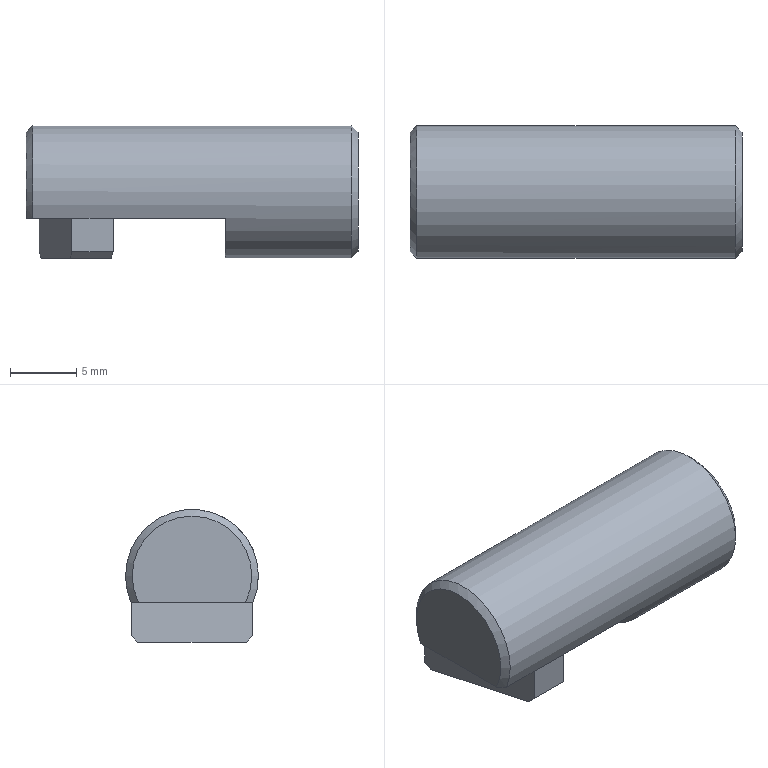Component | NX | GUIDE_PILLAR_B | 1 solid | 15 faces | box 25 x 10 x 10 mm | volume 1745 mm3 | plane 12 | cone 2 | cylinder 1 | commonest cylinder face diameters 10 x1
STEP:
#1=CARTESIAN_POINT('',(0.,0.,0.));
#2=DIRECTION('',(0.,0.,1.));
#3=DIRECTION('',(1.,0.,0.));
#4=AXIS2_PLACEMENT_3D('',#1,#2,#3);
#5=CARTESIAN_POINT('',(-78.542,99.583,86.5));
#6=VERTEX_POINT('',#5);
#7=CARTESIAN_POINT('',(-76.086,90.417,86.5));
#8=VERTEX_POINT('',#7);
#9=CARTESIAN_POINT('',(-78.542,99.583,86.5));
#10=DIRECTION('',(0.2588,-0.9659,0.));
#11=VECTOR('',#10,1.);
#12=LINE('',#9,#11);
#13=CARTESIAN_POINT('',(-67.647,89.2,86.5));
#14=DIRECTION('',(0.,0.,1.));
#15=DIRECTION('',(1.,0.,0.));
#16=AXIS2_PLACEMENT_3D('',#13,#14,#15);
#17=PLANE('',#16);
#18=CARTESIAN_POINT('',(-10.894,10.383));
#19=DIRECTION('',(0.2588,-0.9659));
#20=VECTOR('',#19,1.);
#21=LINE('',#18,#20);
#22=(GEOMETRIC_REPRESENTATION_CONTEXT(2)PARAMETRIC_REPRESENTATION_CONTEXT()REPRESENTATION_CONTEXT('',''));
#23=DEFINITIONAL_REPRESENTATION('',(#21),#22);
#24=PCURVE('',#17,#23);
#25=CARTESIAN_POINT('',(-78.542,99.583,83.5));
#26=DIRECTION('',(-0.9659,-0.2588,0.));
#27=DIRECTION('',(0.2588,-0.9659,0.));
#28=AXIS2_PLACEMENT_3D('',#25,#26,#27);
#29=PLANE('',#28);
#30=CARTESIAN_POINT('',(0.,3.));
#31=DIRECTION('',(1.,0.));
#32=VECTOR('',#31,1.);
#33=LINE('',#30,#32);
#34=(GEOMETRIC_REPRESENTATION_CONTEXT(2)PARAMETRIC_REPRESENTATION_CONTEXT()REPRESENTATION_CONTEXT('',''));
#35=DEFINITIONAL_REPRESENTATION('',(#33),#34);
#36=PCURVE('',#29,#35);
#37=SURFACE_CURVE('',#12,(#24,#36),.PCURVE_S1.);
#38=EDGE_CURVE('',#6,#8,#37,.T.);
#39=ORIENTED_EDGE('',*,*,#38,.F.);
#40=CARTESIAN_POINT('',(-67.647,99.583,86.5));
#41=VERTEX_POINT('',#40);
#42=CARTESIAN_POINT('',(-82.647,99.583,86.5));
#43=DIRECTION('',(1.,0.,0.));
#44=VECTOR('',#43,1.);
#45=LINE('',#42,#44);
#46=CARTESIAN_POINT('',(-15.,10.383));
#47=DIRECTION('',(1.,0.));
#48=VECTOR('',#47,1.);
#49=LINE('',#46,#48);
#50=(GEOMETRIC_REPRESENTATION_CONTEXT(2)PARAMETRIC_REPRESENTATION_CONTEXT()REPRESENTATION_CONTEXT('',''));
#51=DEFINITIONAL_REPRESENTATION('',(#49),#50);
#52=PCURVE('',#17,#51);
#53=CARTESIAN_POINT('',(-82.647,95.,88.5));
#54=DIRECTION('',(1.,0.,0.));
#55=DIRECTION('',(0.,1.,0.));
#56=AXIS2_PLACEMENT_3D('',#53,#54,#55);
#57=CYLINDRICAL_SURFACE('',#56,5.);
#58=CARTESIAN_POINT('',(5.872,0.));
#59=DIRECTION('',(0.,1.));
#60=VECTOR('',#59,1.);
#61=LINE('',#58,#60);
#62=(GEOMETRIC_REPRESENTATION_CONTEXT(2)PARAMETRIC_REPRESENTATION_CONTEXT()REPRESENTATION_CONTEXT('',''));
#63=DEFINITIONAL_REPRESENTATION('',(#61),#62);
#64=PCURVE('',#57,#63);
#65=SURFACE_CURVE('',#45,(#52,#64),.PCURVE_S1.);
#66=EDGE_CURVE('',#6,#41,#65,.T.);
#67=ORIENTED_EDGE('',*,*,#66,.T.);
#68=CARTESIAN_POINT('',(-67.647,90.417,86.5));
#69=VERTEX_POINT('',#68);
#70=CARTESIAN_POINT('',(-67.647,89.2,86.5));
#71=DIRECTION('',(0.,-1.,0.));
#72=VECTOR('',#71,1.);
#73=LINE('',#70,#72);
#74=CARTESIAN_POINT('',(0.,0.));
#75=DIRECTION('',(0.,-1.));
#76=VECTOR('',#75,1.);
#77=LINE('',#74,#76);
#78=(GEOMETRIC_REPRESENTATION_CONTEXT(2)PARAMETRIC_REPRESENTATION_CONTEXT()REPRESENTATION_CONTEXT('',''));
#79=DEFINITIONAL_REPRESENTATION('',(#77),#78);
#80=PCURVE('',#17,#79);
#81=CARTESIAN_POINT('',(-67.647,95.,88.5));
#82=DIRECTION('',(-1.,0.,0.));
#83=DIRECTION('',(0.,-1.,0.));
#84=AXIS2_PLACEMENT_3D('',#81,#82,#83);
#85=PLANE('',#84);
#86=CARTESIAN_POINT('',(5.8,-2.));
#87=DIRECTION('',(1.,0.));
#88=VECTOR('',#87,1.);
#89=LINE('',#86,#88);
#90=(GEOMETRIC_REPRESENTATION_CONTEXT(2)PARAMETRIC_REPRESENTATION_CONTEXT()REPRESENTATION_CONTEXT('',''));
#91=DEFINITIONAL_REPRESENTATION('',(#89),#90);
#92=PCURVE('',#85,#91);
#93=SURFACE_CURVE('',#73,(#80,#92),.PCURVE_S1.);
#94=EDGE_CURVE('',#41,#69,#93,.T.);
#95=ORIENTED_EDGE('',*,*,#94,.T.);
#96=CARTESIAN_POINT('',(-82.647,90.417,86.5));
#97=DIRECTION('',(-1.,0.,0.));
#98=VECTOR('',#97,1.);
#99=LINE('',#96,#98);
#100=CARTESIAN_POINT('',(-15.,1.217));
#101=DIRECTION('',(-1.,0.));
#102=VECTOR('',#101,1.);
#103=LINE('',#100,#102);
#104=(GEOMETRIC_REPRESENTATION_CONTEXT(2)PARAMETRIC_REPRESENTATION_CONTEXT()REPRESENTATION_CONTEXT('',''));
#105=DEFINITIONAL_REPRESENTATION('',(#103),#104);
#106=PCURVE('',#17,#105);
#107=CARTESIAN_POINT('',(3.553,0.));
#108=DIRECTION('',(0.,-1.));
#109=VECTOR('',#108,1.);
#110=LINE('',#107,#109);
#111=(GEOMETRIC_REPRESENTATION_CONTEXT(2)PARAMETRIC_REPRESENTATION_CONTEXT()REPRESENTATION_CONTEXT('',''));
#112=DEFINITIONAL_REPRESENTATION('',(#110),#111);
#113=PCURVE('',#57,#112);
#114=SURFACE_CURVE('',#99,(#106,#113),.PCURVE_S1.);
#115=EDGE_CURVE('',#69,#8,#114,.T.);
#116=ORIENTED_EDGE('',*,*,#115,.T.);
#117=EDGE_LOOP('',(#39,#67,#95,#116));
#118=FACE_BOUND('',#117,.T.);
#119=ADVANCED_FACE('',(#118),#17,.F.);
#120=CARTESIAN_POINT('',(-79.192,90.417,86.5));
#121=VERTEX_POINT('',#120);
#122=CARTESIAN_POINT('',(-81.647,99.583,86.5));
#123=VERTEX_POINT('',#122);
#124=CARTESIAN_POINT('',(-79.192,90.417,86.5));
#125=DIRECTION('',(-0.2588,0.9659,0.));
#126=VECTOR('',#125,1.);
#127=LINE('',#124,#126);
#128=CARTESIAN_POINT('',(-67.647,89.2,86.5));
#129=DIRECTION('',(0.,0.,1.));
#130=DIRECTION('',(1.,0.,0.));
#131=AXIS2_PLACEMENT_3D('',#128,#129,#130);
#132=PLANE('',#131);
#133=CARTESIAN_POINT('',(-11.544,1.217));
#134=DIRECTION('',(-0.2588,0.9659));
#135=VECTOR('',#134,1.);
#136=LINE('',#133,#135);
#137=(GEOMETRIC_REPRESENTATION_CONTEXT(2)PARAMETRIC_REPRESENTATION_CONTEXT()REPRESENTATION_CONTEXT('',''));
#138=DEFINITIONAL_REPRESENTATION('',(#136),#137);
#139=PCURVE('',#132,#138);
#140=CARTESIAN_POINT('',(-79.192,90.417,83.5));
#141=DIRECTION('',(0.9659,0.2588,0.));
#142=DIRECTION('',(-0.2588,0.9659,0.));
#143=AXIS2_PLACEMENT_3D('',#140,#141,#142);
#144=PLANE('',#143);
#145=CARTESIAN_POINT('',(0.,3.));
#146=DIRECTION('',(1.,0.));
#147=VECTOR('',#146,1.);
#148=LINE('',#145,#147);
#149=(GEOMETRIC_REPRESENTATION_CONTEXT(2)PARAMETRIC_REPRESENTATION_CONTEXT()REPRESENTATION_CONTEXT('',''));
#150=DEFINITIONAL_REPRESENTATION('',(#148),#149);
#151=PCURVE('',#144,#150);
#152=SURFACE_CURVE('',#127,(#139,#151),.PCURVE_S1.);
#153=EDGE_CURVE('',#121,#123,#152,.T.);
#154=ORIENTED_EDGE('',*,*,#153,.F.);
#155=CARTESIAN_POINT('',(-82.147,90.417,86.5));
#156=VERTEX_POINT('',#155);
#157=CARTESIAN_POINT('',(-82.647,90.417,86.5));
#158=DIRECTION('',(-1.,0.,0.));
#159=VECTOR('',#158,1.);
#160=LINE('',#157,#159);
#161=CARTESIAN_POINT('',(-15.,1.217));
#162=DIRECTION('',(-1.,0.));
#163=VECTOR('',#162,1.);
#164=LINE('',#161,#163);
#165=(GEOMETRIC_REPRESENTATION_CONTEXT(2)PARAMETRIC_REPRESENTATION_CONTEXT()REPRESENTATION_CONTEXT('',''));
#166=DEFINITIONAL_REPRESENTATION('',(#164),#165);
#167=PCURVE('',#132,#166);
#168=CARTESIAN_POINT('',(3.553,0.));
#169=DIRECTION('',(0.,-1.));
#170=VECTOR('',#169,1.);
#171=LINE('',#168,#170);
#172=(GEOMETRIC_REPRESENTATION_CONTEXT(2)PARAMETRIC_REPRESENTATION_CONTEXT()REPRESENTATION_CONTEXT('',''));
#173=DEFINITIONAL_REPRESENTATION('',(#171),#172);
#174=PCURVE('',#57,#173);
#175=SURFACE_CURVE('',#160,(#167,#174),.PCURVE_S1.);
#176=EDGE_CURVE('',#121,#156,#175,.T.);
#177=ORIENTED_EDGE('',*,*,#176,.T.);
#178=CARTESIAN_POINT('',(-82.647,90.969,86.5));
#179=VERTEX_POINT('',#178);
#180=CARTESIAN_POINT('',(-82.147,90.417,86.5));
#181=CARTESIAN_POINT('',(-82.315,90.6,86.5));
#182=CARTESIAN_POINT('',(-82.482,90.784,86.5));
#183=CARTESIAN_POINT('',(-82.647,90.969,86.5));
#184=B_SPLINE_CURVE_WITH_KNOTS('',3,(#180,#181,#182,#183),.UNSPECIFIED.,.F.,.F.,(4,4),(0.,1.),.PIECEWISE_BEZIER_KNOTS.);
#185=CARTESIAN_POINT('',(-14.5,1.217));
#186=CARTESIAN_POINT('',(-14.668,1.4));
#187=CARTESIAN_POINT('',(-14.834,1.584));
#188=CARTESIAN_POINT('',(-15.,1.769));
#189=B_SPLINE_CURVE_WITH_KNOTS('',3,(#185,#186,#187,#188),.UNSPECIFIED.,.F.,.F.,(4,4),(0.,1.),.PIECEWISE_BEZIER_KNOTS.);
#190=(GEOMETRIC_REPRESENTATION_CONTEXT(2)PARAMETRIC_REPRESENTATION_CONTEXT()REPRESENTATION_CONTEXT('',''));
#191=DEFINITIONAL_REPRESENTATION('',(#189),#190);
#192=PCURVE('',#132,#191);
#193=CARTESIAN_POINT('',(-82.147,95.,88.5));
#194=DIRECTION('',(1.,0.,0.));
#195=DIRECTION('',(0.,1.,0.));
#196=AXIS2_PLACEMENT_3D('',#193,#194,#195);
#197=CONICAL_SURFACE('',#196,5.,0.7854);
#198=CARTESIAN_POINT('',(3.553,-0.));
#199=CARTESIAN_POINT('',(3.602,-0.5));
#200=B_SPLINE_CURVE_WITH_KNOTS('',1,(#198,#199),.UNSPECIFIED.,.F.,.F.,(2,2),(0.,1.),.PIECEWISE_BEZIER_KNOTS.);
#201=(GEOMETRIC_REPRESENTATION_CONTEXT(2)PARAMETRIC_REPRESENTATION_CONTEXT()REPRESENTATION_CONTEXT('',''));
#202=DEFINITIONAL_REPRESENTATION('',(#200),#201);
#203=PCURVE('',#197,#202);
#204=SURFACE_CURVE('',#184,(#192,#203),.PCURVE_S1.);
#205=EDGE_CURVE('',#156,#179,#204,.T.);
#206=ORIENTED_EDGE('',*,*,#205,.T.);
#207=CARTESIAN_POINT('',(-82.647,99.031,86.5));
#208=VERTEX_POINT('',#207);
#209=CARTESIAN_POINT('',(-82.647,89.2,86.5));
#210=DIRECTION('',(0.,1.,0.));
#211=VECTOR('',#210,1.);
#212=LINE('',#209,#211);
#213=CARTESIAN_POINT('',(-15.,0.));
#214=DIRECTION('',(0.,1.));
#215=VECTOR('',#214,1.);
#216=LINE('',#213,#215);
#217=(GEOMETRIC_REPRESENTATION_CONTEXT(2)PARAMETRIC_REPRESENTATION_CONTEXT()REPRESENTATION_CONTEXT('',''));
#218=DEFINITIONAL_REPRESENTATION('',(#216),#217);
#219=PCURVE('',#132,#218);
#220=CARTESIAN_POINT('',(-82.647,95.,88.5));
#221=DIRECTION('',(-1.,0.,0.));
#222=DIRECTION('',(0.,-1.,0.));
#223=AXIS2_PLACEMENT_3D('',#220,#221,#222);
#224=PLANE('',#223);
#225=CARTESIAN_POINT('',(5.8,-2.));
#226=DIRECTION('',(-1.,0.));
#227=VECTOR('',#226,1.);
#228=LINE('',#225,#227);
#229=(GEOMETRIC_REPRESENTATION_CONTEXT(2)PARAMETRIC_REPRESENTATION_CONTEXT()REPRESENTATION_CONTEXT('',''));
#230=DEFINITIONAL_REPRESENTATION('',(#228),#229);
#231=PCURVE('',#224,#230);
#232=SURFACE_CURVE('',#212,(#219,#231),.PCURVE_S1.);
#233=EDGE_CURVE('',#179,#208,#232,.T.);
#234=ORIENTED_EDGE('',*,*,#233,.T.);
#235=CARTESIAN_POINT('',(-82.147,99.583,86.5));
#236=VERTEX_POINT('',#235);
#237=CARTESIAN_POINT('',(-82.647,99.031,86.5));
#238=CARTESIAN_POINT('',(-82.482,99.216,86.5));
#239=CARTESIAN_POINT('',(-82.315,99.4,86.5));
#240=CARTESIAN_POINT('',(-82.147,99.583,86.5));
#241=B_SPLINE_CURVE_WITH_KNOTS('',3,(#237,#238,#239,#240),.UNSPECIFIED.,.F.,.F.,(4,4),(0.,1.),.PIECEWISE_BEZIER_KNOTS.);
#242=CARTESIAN_POINT('',(-15.,9.831));
#243=CARTESIAN_POINT('',(-14.834,10.016));
#244=CARTESIAN_POINT('',(-14.668,10.2));
#245=CARTESIAN_POINT('',(-14.5,10.383));
#246=B_SPLINE_CURVE_WITH_KNOTS('',3,(#242,#243,#244,#245),.UNSPECIFIED.,.F.,.F.,(4,4),(0.,1.),.PIECEWISE_BEZIER_KNOTS.);
#247=(GEOMETRIC_REPRESENTATION_CONTEXT(2)PARAMETRIC_REPRESENTATION_CONTEXT()REPRESENTATION_CONTEXT('',''));
#248=DEFINITIONAL_REPRESENTATION('',(#246),#247);
#249=PCURVE('',#132,#248);
#250=CARTESIAN_POINT('',(-0.4606,-0.5));
#251=CARTESIAN_POINT('',(-0.4115,-0.));
#252=B_SPLINE_CURVE_WITH_KNOTS('',1,(#250,#251),.UNSPECIFIED.,.F.,.F.,(2,2),(0.,1.),.PIECEWISE_BEZIER_KNOTS.);
#253=(GEOMETRIC_REPRESENTATION_CONTEXT(2)PARAMETRIC_REPRESENTATION_CONTEXT()REPRESENTATION_CONTEXT('',''));
#254=DEFINITIONAL_REPRESENTATION('',(#252),#253);
#255=PCURVE('',#197,#254);
#256=SURFACE_CURVE('',#241,(#249,#255),.PCURVE_S1.);
#257=EDGE_CURVE('',#208,#236,#256,.T.);
#258=ORIENTED_EDGE('',*,*,#257,.T.);
#259=CARTESIAN_POINT('',(-82.647,99.583,86.5));
#260=DIRECTION('',(1.,0.,0.));
#261=VECTOR('',#260,1.);
#262=LINE('',#259,#261);
#263=CARTESIAN_POINT('',(-15.,10.383));
#264=DIRECTION('',(1.,0.));
#265=VECTOR('',#264,1.);
#266=LINE('',#263,#265);
#267=(GEOMETRIC_REPRESENTATION_CONTEXT(2)PARAMETRIC_REPRESENTATION_CONTEXT()REPRESENTATION_CONTEXT('',''));
#268=DEFINITIONAL_REPRESENTATION('',(#266),#267);
#269=PCURVE('',#132,#268);
#270=CARTESIAN_POINT('',(5.872,0.));
#271=DIRECTION('',(0.,1.));
#272=VECTOR('',#271,1.);
#273=LINE('',#270,#272);
#274=(GEOMETRIC_REPRESENTATION_CONTEXT(2)PARAMETRIC_REPRESENTATION_CONTEXT()REPRESENTATION_CONTEXT('',''));
#275=DEFINITIONAL_REPRESENTATION('',(#273),#274);
#276=PCURVE('',#57,#275);
#277=SURFACE_CURVE('',#262,(#269,#276),.PCURVE_S1.);
#278=EDGE_CURVE('',#236,#123,#277,.T.);
#279=ORIENTED_EDGE('',*,*,#278,.T.);
#280=EDGE_LOOP('',(#154,#177,#206,#234,#258,#279));
#281=FACE_BOUND('',#280,.T.);
#282=ADVANCED_FACE('',(#281),#132,.F.);
#283=CARTESIAN_POINT('',(-57.647,99.5,88.5));
#284=VERTEX_POINT('',#283);
#285=CARTESIAN_POINT('',(-57.647,95.,88.5));
#286=DIRECTION('',(1.,0.,0.));
#287=DIRECTION('',(0.,1.,0.));
#288=AXIS2_PLACEMENT_3D('',#285,#286,#287);
#289=CIRCLE('',#288,4.5);
#290=CARTESIAN_POINT('',(-57.647,95.,88.5));
#291=DIRECTION('',(1.,0.,0.));
#292=DIRECTION('',(0.,1.,0.));
#293=AXIS2_PLACEMENT_3D('',#290,#291,#292);
#294=PLANE('',#293);
#295=CARTESIAN_POINT('',(0.,0.));
#296=DIRECTION('',(1.,0.));
#297=AXIS2_PLACEMENT_2D('',#295,#296);
#298=CIRCLE('',#297,4.5);
#299=(GEOMETRIC_REPRESENTATION_CONTEXT(2)PARAMETRIC_REPRESENTATION_CONTEXT()REPRESENTATION_CONTEXT('',''));
#300=DEFINITIONAL_REPRESENTATION('',(#298),#299);
#301=PCURVE('',#294,#300);
#302=CARTESIAN_POINT('',(-58.147,95.,88.5));
#303=DIRECTION('',(-1.,0.,0.));
#304=DIRECTION('',(0.,-1.,0.));
#305=AXIS2_PLACEMENT_3D('',#302,#303,#304);
#306=CONICAL_SURFACE('',#305,5.,0.7854);
#307=CARTESIAN_POINT('',(9.425,-0.5));
#308=DIRECTION('',(-1.,0.));
#309=VECTOR('',#308,1.);
#310=LINE('',#307,#309);
#311=(GEOMETRIC_REPRESENTATION_CONTEXT(2)PARAMETRIC_REPRESENTATION_CONTEXT()REPRESENTATION_CONTEXT('',''));
#312=DEFINITIONAL_REPRESENTATION('',(#310),#311);
#313=PCURVE('',#306,#312);
#314=SURFACE_CURVE('',#289,(#301,#313),.PCURVE_S1.);
#315=EDGE_CURVE('',#284,#284,#314,.T.);
#316=ORIENTED_EDGE('',*,*,#315,.T.);
#317=EDGE_LOOP('',(#316));
#318=FACE_BOUND('',#317,.T.);
#319=ADVANCED_FACE('',(#318),#294,.T.);
#320=ORIENTED_EDGE('',*,*,#233,.F.);
#321=CARTESIAN_POINT('',(-82.647,95.,88.5));
#322=DIRECTION('',(-1.,0.,0.));
#323=DIRECTION('',(0.,-1.,0.));
#324=AXIS2_PLACEMENT_3D('',#321,#322,#323);
#325=CIRCLE('',#324,4.5);
#326=CARTESIAN_POINT('',(0.,0.));
#327=DIRECTION('',(1.,0.));
#328=AXIS2_PLACEMENT_2D('',#326,#327);
#329=CIRCLE('',#328,4.5);
#330=(GEOMETRIC_REPRESENTATION_CONTEXT(2)PARAMETRIC_REPRESENTATION_CONTEXT()REPRESENTATION_CONTEXT('',''));
#331=DEFINITIONAL_REPRESENTATION('',(#329),#330);
#332=PCURVE('',#224,#331);
#333=CARTESIAN_POINT('',(9.425,-0.5));
#334=DIRECTION('',(-1.,0.));
#335=VECTOR('',#334,1.);
#336=LINE('',#333,#335);
#337=(GEOMETRIC_REPRESENTATION_CONTEXT(2)PARAMETRIC_REPRESENTATION_CONTEXT()REPRESENTATION_CONTEXT('',''));
#338=DEFINITIONAL_REPRESENTATION('',(#336),#337);
#339=PCURVE('',#197,#338);
#340=SURFACE_CURVE('',#325,(#332,#339),.PCURVE_S1.);
#341=EDGE_CURVE('',#179,#208,#340,.T.);
#342=ORIENTED_EDGE('',*,*,#341,.T.);
#343=EDGE_LOOP('',(#320,#342));
#344=FACE_BOUND('',#343,.T.);
#345=ADVANCED_FACE('',(#344),#224,.T.);
#346=ORIENTED_EDGE('',*,*,#115,.F.);
#347=CARTESIAN_POINT('',(-67.647,95.,88.5));
#348=DIRECTION('',(1.,0.,0.));
#349=DIRECTION('',(0.,-1.,0.));
#350=AXIS2_PLACEMENT_3D('',#347,#348,#349);
#351=CIRCLE('',#350,5.);
#352=CARTESIAN_POINT('',(3.142,15.));
#353=DIRECTION('',(1.,0.));
#354=VECTOR('',#353,1.);
#355=LINE('',#352,#354);
#356=(GEOMETRIC_REPRESENTATION_CONTEXT(2)PARAMETRIC_REPRESENTATION_CONTEXT()REPRESENTATION_CONTEXT('',''));
#357=DEFINITIONAL_REPRESENTATION('',(#355),#356);
#358=PCURVE('',#57,#357);
#359=CARTESIAN_POINT('',(5.,0.));
#360=CARTESIAN_POINT('',(5.,-8.66));
#361=CARTESIAN_POINT('',(-2.5,-4.33));
#362=CARTESIAN_POINT('',(-10.,-0.));
#363=CARTESIAN_POINT('',(-2.5,4.33));
#364=CARTESIAN_POINT('',(5.,8.66));
#365=CARTESIAN_POINT('',(5.,0.));
#366=(BOUNDED_CURVE()B_SPLINE_CURVE(2,(#359,#360,#361,#362,#363,#364,#365),.UNSPECIFIED.,.T.,.F.)B_SPLINE_CURVE_WITH_KNOTS((1,2,2,2,2,1),(-2.094,0.,2.094,4.189,6.283,8.378),.UNSPECIFIED.)CURVE()GEOMETRIC_REPRESENTATION_ITEM()RATIONAL_B_SPLINE_CURVE((1.,0.5,1.,0.5,1.,0.5,1.))REPRESENTATION_ITEM(''));
#367=(GEOMETRIC_REPRESENTATION_CONTEXT(2)PARAMETRIC_REPRESENTATION_CONTEXT()REPRESENTATION_CONTEXT('',''));
#368=DEFINITIONAL_REPRESENTATION('',(#366),#367);
#369=PCURVE('',#85,#368);
#370=SURFACE_CURVE('',#351,(#358,#369),.PCURVE_S1.);
#371=EDGE_CURVE('',#69,#41,#370,.T.);
#372=ORIENTED_EDGE('',*,*,#371,.T.);
#373=ORIENTED_EDGE('',*,*,#66,.F.);
#374=CARTESIAN_POINT('',(-81.647,99.583,86.5));
#375=DIRECTION('',(1.,0.,0.));
#376=VECTOR('',#375,1.);
#377=LINE('',#374,#376);
#378=CARTESIAN_POINT('',(5.872,1.));
#379=DIRECTION('',(0.,1.));
#380=VECTOR('',#379,1.);
#381=LINE('',#378,#380);
#382=(GEOMETRIC_REPRESENTATION_CONTEXT(2)PARAMETRIC_REPRESENTATION_CONTEXT()REPRESENTATION_CONTEXT('',''));
#383=DEFINITIONAL_REPRESENTATION('',(#381),#382);
#384=PCURVE('',#57,#383);
#385=CARTESIAN_POINT('',(-81.647,99.583,83.5));
#386=DIRECTION('',(0.,-1.,0.));
#387=DIRECTION('',(1.,0.,0.));
#388=AXIS2_PLACEMENT_3D('',#385,#386,#387);
#389=PLANE('',#388);
#390=CARTESIAN_POINT('',(0.,3.));
#391=DIRECTION('',(1.,0.));
#392=VECTOR('',#391,1.);
#393=LINE('',#390,#392);
#394=(GEOMETRIC_REPRESENTATION_CONTEXT(2)PARAMETRIC_REPRESENTATION_CONTEXT()REPRESENTATION_CONTEXT('',''));
#395=DEFINITIONAL_REPRESENTATION('',(#393),#394);
#396=PCURVE('',#389,#395);
#397=SURFACE_CURVE('',#377,(#384,#396),.PCURVE_S1.);
#398=EDGE_CURVE('',#123,#6,#397,.T.);
#399=ORIENTED_EDGE('',*,*,#398,.F.);
#400=ORIENTED_EDGE('',*,*,#278,.F.);
#401=CARTESIAN_POINT('',(-82.147,100.,88.5));
#402=VERTEX_POINT('',#401);
#403=CARTESIAN_POINT('',(-82.147,95.,88.5));
#404=DIRECTION('',(1.,0.,0.));
#405=DIRECTION('',(0.,-1.,0.));
#406=AXIS2_PLACEMENT_3D('',#403,#404,#405);
#407=CIRCLE('',#406,5.);
#408=CARTESIAN_POINT('',(3.142,0.5));
#409=DIRECTION('',(1.,0.));
#410=VECTOR('',#409,1.);
#411=LINE('',#408,#410);
#412=(GEOMETRIC_REPRESENTATION_CONTEXT(2)PARAMETRIC_REPRESENTATION_CONTEXT()REPRESENTATION_CONTEXT('',''));
#413=DEFINITIONAL_REPRESENTATION('',(#411),#412);
#414=PCURVE('',#57,#413);
#415=CARTESIAN_POINT('',(-3.142,0.));
#416=DIRECTION('',(1.,-0.));
#417=VECTOR('',#416,1.);
#418=LINE('',#415,#417);
#419=(GEOMETRIC_REPRESENTATION_CONTEXT(2)PARAMETRIC_REPRESENTATION_CONTEXT()REPRESENTATION_CONTEXT('',''));
#420=DEFINITIONAL_REPRESENTATION('',(#418),#419);
#421=PCURVE('',#197,#420);
#422=SURFACE_CURVE('',#407,(#414,#421),.PCURVE_S1.);
#423=EDGE_CURVE('',#236,#402,#422,.T.);
#424=ORIENTED_EDGE('',*,*,#423,.T.);
#425=CARTESIAN_POINT('',(-58.147,100.,88.5));
#426=VERTEX_POINT('',#425);
#427=CARTESIAN_POINT('',(-82.147,100.,88.5));
#428=CARTESIAN_POINT('',(-58.147,100.,88.5));
#429=B_SPLINE_CURVE_WITH_KNOTS('',1,(#427,#428),.UNSPECIFIED.,.F.,.F.,(2,2),(0.5,24.5),.PIECEWISE_BEZIER_KNOTS.);
#430=CARTESIAN_POINT('',(6.283,0.));
#431=DIRECTION('',(0.,1.));
#432=VECTOR('',#431,1.);
#433=LINE('',#430,#432);
#434=(GEOMETRIC_REPRESENTATION_CONTEXT(2)PARAMETRIC_REPRESENTATION_CONTEXT()REPRESENTATION_CONTEXT('',''));
#435=DEFINITIONAL_REPRESENTATION('',(#433),#434);
#436=PCURVE('',#57,#435);
#437=CARTESIAN_POINT('',(0.,0.));
#438=DIRECTION('',(0.,1.));
#439=VECTOR('',#438,1.);
#440=LINE('',#437,#439);
#441=(GEOMETRIC_REPRESENTATION_CONTEXT(2)PARAMETRIC_REPRESENTATION_CONTEXT()REPRESENTATION_CONTEXT('',''));
#442=DEFINITIONAL_REPRESENTATION('',(#440),#441);
#443=PCURVE('',#57,#442);
#444=SEAM_CURVE('',#429,(#436,#443),.PCURVE_S1.);
#445=EDGE_CURVE('',#402,#426,#444,.T.);
#446=ORIENTED_EDGE('',*,*,#445,.T.);
#447=CARTESIAN_POINT('',(-58.147,95.,88.5));
#448=DIRECTION('',(-1.,0.,0.));
#449=DIRECTION('',(0.,1.,0.));
#450=AXIS2_PLACEMENT_3D('',#447,#448,#449);
#451=CIRCLE('',#450,5.);
#452=CARTESIAN_POINT('',(6.283,24.5));
#453=DIRECTION('',(-1.,0.));
#454=VECTOR('',#453,1.);
#455=LINE('',#452,#454);
#456=(GEOMETRIC_REPRESENTATION_CONTEXT(2)PARAMETRIC_REPRESENTATION_CONTEXT()REPRESENTATION_CONTEXT('',''));
#457=DEFINITIONAL_REPRESENTATION('',(#455),#456);
#458=PCURVE('',#57,#457);
#459=CARTESIAN_POINT('',(3.142,0.));
#460=DIRECTION('',(1.,0.));
#461=VECTOR('',#460,1.);
#462=LINE('',#459,#461);
#463=(GEOMETRIC_REPRESENTATION_CONTEXT(2)PARAMETRIC_REPRESENTATION_CONTEXT()REPRESENTATION_CONTEXT('',''));
#464=DEFINITIONAL_REPRESENTATION('',(#462),#463);
#465=PCURVE('',#306,#464);
#466=SURFACE_CURVE('',#451,(#458,#465),.PCURVE_S1.);
#467=EDGE_CURVE('',#426,#426,#466,.T.);
#468=ORIENTED_EDGE('',*,*,#467,.T.);
#469=ORIENTED_EDGE('',*,*,#445,.F.);
#470=CARTESIAN_POINT('',(-82.147,95.,88.5));
#471=DIRECTION('',(1.,0.,0.));
#472=DIRECTION('',(0.,-1.,0.));
#473=AXIS2_PLACEMENT_3D('',#470,#471,#472);
#474=CIRCLE('',#473,5.);
#475=CARTESIAN_POINT('',(-3.142,0.5));
#476=DIRECTION('',(1.,0.));
#477=VECTOR('',#476,1.);
#478=LINE('',#475,#477);
#479=(GEOMETRIC_REPRESENTATION_CONTEXT(2)PARAMETRIC_REPRESENTATION_CONTEXT()REPRESENTATION_CONTEXT('',''));
#480=DEFINITIONAL_REPRESENTATION('',(#478),#479);
#481=PCURVE('',#57,#480);
#482=CARTESIAN_POINT('',(-3.142,0.));
#483=DIRECTION('',(1.,-0.));
#484=VECTOR('',#483,1.);
#485=LINE('',#482,#484);
#486=(GEOMETRIC_REPRESENTATION_CONTEXT(2)PARAMETRIC_REPRESENTATION_CONTEXT()REPRESENTATION_CONTEXT('',''));
#487=DEFINITIONAL_REPRESENTATION('',(#485),#486);
#488=PCURVE('',#197,#487);
#489=SURFACE_CURVE('',#474,(#481,#488),.PCURVE_S1.);
#490=EDGE_CURVE('',#402,#156,#489,.T.);
#491=ORIENTED_EDGE('',*,*,#490,.T.);
#492=ORIENTED_EDGE('',*,*,#176,.F.);
#493=CARTESIAN_POINT('',(-76.086,90.417,86.5));
#494=DIRECTION('',(-1.,0.,0.));
#495=VECTOR('',#494,1.);
#496=LINE('',#493,#495);
#497=CARTESIAN_POINT('',(3.553,6.562));
#498=DIRECTION('',(0.,-1.));
#499=VECTOR('',#498,1.);
#500=LINE('',#497,#499);
#501=(GEOMETRIC_REPRESENTATION_CONTEXT(2)PARAMETRIC_REPRESENTATION_CONTEXT()REPRESENTATION_CONTEXT('',''));
#502=DEFINITIONAL_REPRESENTATION('',(#500),#501);
#503=PCURVE('',#57,#502);
#504=CARTESIAN_POINT('',(-76.086,90.417,83.5));
#505=DIRECTION('',(0.,1.,0.));
#506=DIRECTION('',(-1.,0.,0.));
#507=AXIS2_PLACEMENT_3D('',#504,#505,#506);
#508=PLANE('',#507);
#509=CARTESIAN_POINT('',(0.,3.));
#510=DIRECTION('',(1.,0.));
#511=VECTOR('',#510,1.);
#512=LINE('',#509,#511);
#513=(GEOMETRIC_REPRESENTATION_CONTEXT(2)PARAMETRIC_REPRESENTATION_CONTEXT()REPRESENTATION_CONTEXT('',''));
#514=DEFINITIONAL_REPRESENTATION('',(#512),#513);
#515=PCURVE('',#508,#514);
#516=SURFACE_CURVE('',#496,(#503,#515),.PCURVE_S1.);
#517=EDGE_CURVE('',#8,#121,#516,.T.);
#518=ORIENTED_EDGE('',*,*,#517,.F.);
#519=EDGE_LOOP('',(#346,#372,#373,#399,#400,#424,#446,#468,#469,#491,#492,#518));
#520=FACE_BOUND('',#519,.T.);
#521=ADVANCED_FACE('',(#520),#57,.T.);
#522=ORIENTED_EDGE('',*,*,#205,.F.);
#523=ORIENTED_EDGE('',*,*,#490,.F.);
#524=ORIENTED_EDGE('',*,*,#423,.F.);
#525=ORIENTED_EDGE('',*,*,#257,.F.);
#526=ORIENTED_EDGE('',*,*,#341,.F.);
#527=EDGE_LOOP('',(#522,#523,#524,#525,#526));
#528=FACE_BOUND('',#527,.T.);
#529=ADVANCED_FACE('',(#528),#197,.T.);
#530=ORIENTED_EDGE('',*,*,#315,.F.);
#531=CARTESIAN_POINT('',(-57.647,99.5,88.5));
#532=CARTESIAN_POINT('',(-58.147,100.,88.5));
#533=B_SPLINE_CURVE_WITH_KNOTS('',1,(#531,#532),.UNSPECIFIED.,.F.,.F.,(2,2),(-0.7071,0.),.PIECEWISE_BEZIER_KNOTS.);
#534=CARTESIAN_POINT('',(9.425,0.));
#535=DIRECTION('',(0.,1.));
#536=VECTOR('',#535,1.);
#537=LINE('',#534,#536);
#538=(GEOMETRIC_REPRESENTATION_CONTEXT(2)PARAMETRIC_REPRESENTATION_CONTEXT()REPRESENTATION_CONTEXT('',''));
#539=DEFINITIONAL_REPRESENTATION('',(#537),#538);
#540=PCURVE('',#306,#539);
#541=CARTESIAN_POINT('',(3.142,0.));
#542=DIRECTION('',(0.,1.));
#543=VECTOR('',#542,1.);
#544=LINE('',#541,#543);
#545=(GEOMETRIC_REPRESENTATION_CONTEXT(2)PARAMETRIC_REPRESENTATION_CONTEXT()REPRESENTATION_CONTEXT('',''));
#546=DEFINITIONAL_REPRESENTATION('',(#544),#545);
#547=PCURVE('',#306,#546);
#548=SEAM_CURVE('',#533,(#540,#547),.PCURVE_S1.);
#549=EDGE_CURVE('',#284,#426,#548,.T.);
#550=ORIENTED_EDGE('',*,*,#549,.T.);
#551=ORIENTED_EDGE('',*,*,#467,.F.);
#552=ORIENTED_EDGE('',*,*,#549,.F.);
#553=EDGE_LOOP('',(#530,#550,#551,#552));
#554=FACE_BOUND('',#553,.T.);
#555=ADVANCED_FACE('',(#554),#306,.T.);
#556=ORIENTED_EDGE('',*,*,#94,.F.);
#557=ORIENTED_EDGE('',*,*,#371,.F.);
#558=EDGE_LOOP('',(#556,#557));
#559=FACE_BOUND('',#558,.T.);
#560=ADVANCED_FACE('',(#559),#85,.T.);
#561=CARTESIAN_POINT('',(-78.408,99.083,83.5));
#562=VERTEX_POINT('',#561);
#563=CARTESIAN_POINT('',(-76.22,90.917,83.5));
#564=VERTEX_POINT('',#563);
#565=CARTESIAN_POINT('',(-78.542,99.583,83.5));
#566=DIRECTION('',(0.2588,-0.9659,0.));
#567=VECTOR('',#566,1.);
#568=LINE('',#565,#567);
#569=CARTESIAN_POINT('',(0.,0.));
#570=DIRECTION('',(1.,0.));
#571=VECTOR('',#570,1.);
#572=LINE('',#569,#571);
#573=(GEOMETRIC_REPRESENTATION_CONTEXT(2)PARAMETRIC_REPRESENTATION_CONTEXT()REPRESENTATION_CONTEXT('',''));
#574=DEFINITIONAL_REPRESENTATION('',(#572),#573);
#575=PCURVE('',#29,#574);
#576=CARTESIAN_POINT('',(-82.647,95.,83.5));
#577=DIRECTION('',(0.,0.,-1.));
#578=DIRECTION('',(-1.,0.,0.));
#579=AXIS2_PLACEMENT_3D('',#576,#577,#578);
#580=PLANE('',#579);
#581=CARTESIAN_POINT('',(-4.106,4.583));
#582=DIRECTION('',(-0.2588,-0.9659));
#583=VECTOR('',#582,1.);
#584=LINE('',#581,#583);
#585=(GEOMETRIC_REPRESENTATION_CONTEXT(2)PARAMETRIC_REPRESENTATION_CONTEXT()REPRESENTATION_CONTEXT('',''));
#586=DEFINITIONAL_REPRESENTATION('',(#584),#585);
#587=PCURVE('',#580,#586);
#588=SURFACE_CURVE('',#568,(#575,#587),.PCURVE_S1.);
#589=EDGE_CURVE('',#562,#564,#588,.T.);
#590=ORIENTED_EDGE('',*,*,#589,.F.);
#591=CARTESIAN_POINT('',(-78.542,99.583,84.));
#592=VERTEX_POINT('',#591);
#593=CARTESIAN_POINT('',(-78.554,99.631,84.048));
#594=DIRECTION('',(-0.1862,0.6947,0.6947));
#595=VECTOR('',#594,1.);
#596=LINE('',#593,#595);
#597=CARTESIAN_POINT('',(-0.05005,0.5483));
#598=DIRECTION('',(-0.7193,0.6947));
#599=VECTOR('',#598,1.);
#600=LINE('',#597,#599);
#601=(GEOMETRIC_REPRESENTATION_CONTEXT(2)PARAMETRIC_REPRESENTATION_CONTEXT()REPRESENTATION_CONTEXT('',''));
#602=DEFINITIONAL_REPRESENTATION('',(#600),#601);
#603=PCURVE('',#29,#602);
#604=CARTESIAN_POINT('',(-82.647,99.083,83.5));
#605=DIRECTION('',(0.,0.7071,-0.7071));
#606=DIRECTION('',(-1.,0.,0.));
#607=AXIS2_PLACEMENT_3D('',#604,#605,#606);
#608=PLANE('',#607);
#609=CARTESIAN_POINT('',(-4.093,0.7755));
#610=DIRECTION('',(0.1862,0.9825));
#611=VECTOR('',#610,1.);
#612=LINE('',#609,#611);
#613=(GEOMETRIC_REPRESENTATION_CONTEXT(2)PARAMETRIC_REPRESENTATION_CONTEXT()REPRESENTATION_CONTEXT('',''));
#614=DEFINITIONAL_REPRESENTATION('',(#612),#613);
#615=PCURVE('',#608,#614);
#616=SURFACE_CURVE('',#596,(#603,#615),.PCURVE_S1.);
#617=EDGE_CURVE('',#562,#592,#616,.T.);
#618=ORIENTED_EDGE('',*,*,#617,.T.);
#619=CARTESIAN_POINT('',(-78.542,99.583,83.5));
#620=DIRECTION('',(0.,0.,1.));
#621=VECTOR('',#620,1.);
#622=LINE('',#619,#621);
#623=CARTESIAN_POINT('',(0.,0.));
#624=DIRECTION('',(0.,1.));
#625=VECTOR('',#624,1.);
#626=LINE('',#623,#625);
#627=(GEOMETRIC_REPRESENTATION_CONTEXT(2)PARAMETRIC_REPRESENTATION_CONTEXT()REPRESENTATION_CONTEXT('',''));
#628=DEFINITIONAL_REPRESENTATION('',(#626),#627);
#629=PCURVE('',#29,#628);
#630=CARTESIAN_POINT('',(3.106,0.));
#631=DIRECTION('',(0.,1.));
#632=VECTOR('',#631,1.);
#633=LINE('',#630,#632);
#634=(GEOMETRIC_REPRESENTATION_CONTEXT(2)PARAMETRIC_REPRESENTATION_CONTEXT()REPRESENTATION_CONTEXT('',''));
#635=DEFINITIONAL_REPRESENTATION('',(#633),#634);
#636=PCURVE('',#389,#635);
#637=SURFACE_CURVE('',#622,(#629,#636),.PCURVE_S1.);
#638=EDGE_CURVE('',#592,#6,#637,.T.);
#639=ORIENTED_EDGE('',*,*,#638,.T.);
#640=ORIENTED_EDGE('',*,*,#38,.T.);
#641=CARTESIAN_POINT('',(-76.086,90.417,84.));
#642=VERTEX_POINT('',#641);
#643=CARTESIAN_POINT('',(-76.086,90.417,83.5));
#644=DIRECTION('',(0.,0.,1.));
#645=VECTOR('',#644,1.);
#646=LINE('',#643,#645);
#647=CARTESIAN_POINT('',(9.488,0.));
#648=DIRECTION('',(0.,1.));
#649=VECTOR('',#648,1.);
#650=LINE('',#647,#649);
#651=(GEOMETRIC_REPRESENTATION_CONTEXT(2)PARAMETRIC_REPRESENTATION_CONTEXT()REPRESENTATION_CONTEXT('',''));
#652=DEFINITIONAL_REPRESENTATION('',(#650),#651);
#653=PCURVE('',#29,#652);
#654=CARTESIAN_POINT('',(0.,0.));
#655=DIRECTION('',(0.,1.));
#656=VECTOR('',#655,1.);
#657=LINE('',#654,#656);
#658=(GEOMETRIC_REPRESENTATION_CONTEXT(2)PARAMETRIC_REPRESENTATION_CONTEXT()REPRESENTATION_CONTEXT('',''));
#659=DEFINITIONAL_REPRESENTATION('',(#657),#658);
#660=PCURVE('',#508,#659);
#661=SURFACE_CURVE('',#646,(#653,#660),.PCURVE_S1.);
#662=EDGE_CURVE('',#642,#8,#661,.T.);
#663=ORIENTED_EDGE('',*,*,#662,.F.);
#664=CARTESIAN_POINT('',(-76.442,91.749,82.669));
#665=DIRECTION('',(-0.1862,0.6947,-0.6947));
#666=VECTOR('',#665,1.);
#667=LINE('',#664,#666);
#668=CARTESIAN_POINT('',(8.11,-0.8313));
#669=DIRECTION('',(-0.7193,-0.6947));
#670=VECTOR('',#669,1.);
#671=LINE('',#668,#670);
#672=(GEOMETRIC_REPRESENTATION_CONTEXT(2)PARAMETRIC_REPRESENTATION_CONTEXT()REPRESENTATION_CONTEXT('',''));
#673=DEFINITIONAL_REPRESENTATION('',(#671),#672);
#674=PCURVE('',#29,#673);
#675=CARTESIAN_POINT('',(-82.647,90.917,83.5));
#676=DIRECTION('',(0.,-0.7071,-0.7071));
#677=DIRECTION('',(1.,0.,0.));
#678=AXIS2_PLACEMENT_3D('',#675,#676,#677);
#679=PLANE('',#678);
#680=CARTESIAN_POINT('',(6.205,-1.176));
#681=DIRECTION('',(-0.1862,-0.9825));
#682=VECTOR('',#681,1.);
#683=LINE('',#680,#682);
#684=(GEOMETRIC_REPRESENTATION_CONTEXT(2)PARAMETRIC_REPRESENTATION_CONTEXT()REPRESENTATION_CONTEXT('',''));
#685=DEFINITIONAL_REPRESENTATION('',(#683),#684);
#686=PCURVE('',#679,#685);
#687=SURFACE_CURVE('',#667,(#674,#686),.PCURVE_S1.);
#688=EDGE_CURVE('',#642,#564,#687,.T.);
#689=ORIENTED_EDGE('',*,*,#688,.T.);
#690=EDGE_LOOP('',(#590,#618,#639,#640,#663,#689));
#691=FACE_BOUND('',#690,.T.);
#692=ADVANCED_FACE('',(#691),#29,.F.);
#693=CARTESIAN_POINT('',(-79.192,90.417,84.));
#694=VERTEX_POINT('',#693);
#695=CARTESIAN_POINT('',(-79.192,90.417,83.5));
#696=DIRECTION('',(0.,0.,1.));
#697=VECTOR('',#696,1.);
#698=LINE('',#695,#697);
#699=CARTESIAN_POINT('',(3.106,0.));
#700=DIRECTION('',(0.,1.));
#701=VECTOR('',#700,1.);
#702=LINE('',#699,#701);
#703=(GEOMETRIC_REPRESENTATION_CONTEXT(2)PARAMETRIC_REPRESENTATION_CONTEXT()REPRESENTATION_CONTEXT('',''));
#704=DEFINITIONAL_REPRESENTATION('',(#702),#703);
#705=PCURVE('',#508,#704);
#706=CARTESIAN_POINT('',(0.,0.));
#707=DIRECTION('',(0.,1.));
#708=VECTOR('',#707,1.);
#709=LINE('',#706,#708);
#710=(GEOMETRIC_REPRESENTATION_CONTEXT(2)PARAMETRIC_REPRESENTATION_CONTEXT()REPRESENTATION_CONTEXT('',''));
#711=DEFINITIONAL_REPRESENTATION('',(#709),#710);
#712=PCURVE('',#144,#711);
#713=SURFACE_CURVE('',#698,(#705,#712),.PCURVE_S1.);
#714=EDGE_CURVE('',#694,#121,#713,.T.);
#715=ORIENTED_EDGE('',*,*,#714,.F.);
#716=CARTESIAN_POINT('',(-76.086,90.417,84.));
#717=DIRECTION('',(1.,0.,0.));
#718=VECTOR('',#717,1.);
#719=LINE('',#716,#718);
#720=CARTESIAN_POINT('',(0.,0.5));
#721=DIRECTION('',(-1.,0.));
#722=VECTOR('',#721,1.);
#723=LINE('',#720,#722);
#724=(GEOMETRIC_REPRESENTATION_CONTEXT(2)PARAMETRIC_REPRESENTATION_CONTEXT()REPRESENTATION_CONTEXT('',''));
#725=DEFINITIONAL_REPRESENTATION('',(#723),#724);
#726=PCURVE('',#508,#725);
#727=CARTESIAN_POINT('',(6.562,0.7071));
#728=DIRECTION('',(1.,0.));
#729=VECTOR('',#728,1.);
#730=LINE('',#727,#729);
#731=(GEOMETRIC_REPRESENTATION_CONTEXT(2)PARAMETRIC_REPRESENTATION_CONTEXT()REPRESENTATION_CONTEXT('',''));
#732=DEFINITIONAL_REPRESENTATION('',(#730),#731);
#733=PCURVE('',#679,#732);
#734=SURFACE_CURVE('',#719,(#726,#733),.PCURVE_S1.);
#735=EDGE_CURVE('',#694,#642,#734,.T.);
#736=ORIENTED_EDGE('',*,*,#735,.T.);
#737=ORIENTED_EDGE('',*,*,#662,.T.);
#738=ORIENTED_EDGE('',*,*,#517,.T.);
#739=EDGE_LOOP('',(#715,#736,#737,#738));
#740=FACE_BOUND('',#739,.T.);
#741=ADVANCED_FACE('',(#740),#508,.F.);
#742=CARTESIAN_POINT('',(-81.647,99.583,84.));
#743=VERTEX_POINT('',#742);
#744=CARTESIAN_POINT('',(-81.647,99.583,83.5));
#745=DIRECTION('',(0.,0.,1.));
#746=VECTOR('',#745,1.);
#747=LINE('',#744,#746);
#748=CARTESIAN_POINT('',(9.488,0.));
#749=DIRECTION('',(0.,1.));
#750=VECTOR('',#749,1.);
#751=LINE('',#748,#750);
#752=(GEOMETRIC_REPRESENTATION_CONTEXT(2)PARAMETRIC_REPRESENTATION_CONTEXT()REPRESENTATION_CONTEXT('',''));
#753=DEFINITIONAL_REPRESENTATION('',(#751),#752);
#754=PCURVE('',#144,#753);
#755=CARTESIAN_POINT('',(0.,0.));
#756=DIRECTION('',(0.,1.));
#757=VECTOR('',#756,1.);
#758=LINE('',#755,#757);
#759=(GEOMETRIC_REPRESENTATION_CONTEXT(2)PARAMETRIC_REPRESENTATION_CONTEXT()REPRESENTATION_CONTEXT('',''));
#760=DEFINITIONAL_REPRESENTATION('',(#758),#759);
#761=PCURVE('',#389,#760);
#762=SURFACE_CURVE('',#747,(#754,#761),.PCURVE_S1.);
#763=EDGE_CURVE('',#743,#123,#762,.T.);
#764=ORIENTED_EDGE('',*,*,#763,.F.);
#765=CARTESIAN_POINT('',(-81.513,99.083,83.5));
#766=VERTEX_POINT('',#765);
#767=CARTESIAN_POINT('',(-81.553,99.229,83.647));
#768=DIRECTION('',(0.1862,-0.6947,-0.6947));
#769=VECTOR('',#768,1.);
#770=LINE('',#767,#769);
#771=CARTESIAN_POINT('',(9.123,0.1467));
#772=DIRECTION('',(-0.7193,-0.6947));
#773=VECTOR('',#772,1.);
#774=LINE('',#771,#773);
#775=(GEOMETRIC_REPRESENTATION_CONTEXT(2)PARAMETRIC_REPRESENTATION_CONTEXT()REPRESENTATION_CONTEXT('',''));
#776=DEFINITIONAL_REPRESENTATION('',(#774),#775);
#777=PCURVE('',#144,#776);
#778=CARTESIAN_POINT('',(-1.095,0.2074));
#779=DIRECTION('',(-0.1862,-0.9825));
#780=VECTOR('',#779,1.);
#781=LINE('',#778,#780);
#782=(GEOMETRIC_REPRESENTATION_CONTEXT(2)PARAMETRIC_REPRESENTATION_CONTEXT()REPRESENTATION_CONTEXT('',''));
#783=DEFINITIONAL_REPRESENTATION('',(#781),#782);
#784=PCURVE('',#608,#783);
#785=SURFACE_CURVE('',#770,(#777,#784),.PCURVE_S1.);
#786=EDGE_CURVE('',#743,#766,#785,.T.);
#787=ORIENTED_EDGE('',*,*,#786,.T.);
#788=CARTESIAN_POINT('',(-79.326,90.917,83.5));
#789=VERTEX_POINT('',#788);
#790=CARTESIAN_POINT('',(-79.192,90.417,83.5));
#791=DIRECTION('',(-0.2588,0.9659,0.));
#792=VECTOR('',#791,1.);
#793=LINE('',#790,#792);
#794=CARTESIAN_POINT('',(0.,0.));
#795=DIRECTION('',(1.,0.));
#796=VECTOR('',#795,1.);
#797=LINE('',#794,#796);
#798=(GEOMETRIC_REPRESENTATION_CONTEXT(2)PARAMETRIC_REPRESENTATION_CONTEXT()REPRESENTATION_CONTEXT('',''));
#799=DEFINITIONAL_REPRESENTATION('',(#797),#798);
#800=PCURVE('',#144,#799);
#801=CARTESIAN_POINT('',(-3.456,-4.583));
#802=DIRECTION('',(0.2588,0.9659));
#803=VECTOR('',#802,1.);
#804=LINE('',#801,#803);
#805=(GEOMETRIC_REPRESENTATION_CONTEXT(2)PARAMETRIC_REPRESENTATION_CONTEXT()REPRESENTATION_CONTEXT('',''));
#806=DEFINITIONAL_REPRESENTATION('',(#804),#805);
#807=PCURVE('',#580,#806);
#808=SURFACE_CURVE('',#793,(#800,#807),.PCURVE_S1.);
#809=EDGE_CURVE('',#789,#766,#808,.T.);
#810=ORIENTED_EDGE('',*,*,#809,.F.);
#811=CARTESIAN_POINT('',(-79.441,91.347,83.07));
#812=DIRECTION('',(0.1862,-0.6947,0.6947));
#813=VECTOR('',#812,1.);
#814=LINE('',#811,#813);
#815=CARTESIAN_POINT('',(0.9624,-0.4296));
#816=DIRECTION('',(-0.7193,0.6947));
#817=VECTOR('',#816,1.);
#818=LINE('',#815,#817);
#819=(GEOMETRIC_REPRESENTATION_CONTEXT(2)PARAMETRIC_REPRESENTATION_CONTEXT()REPRESENTATION_CONTEXT('',''));
#820=DEFINITIONAL_REPRESENTATION('',(#818),#819);
#821=PCURVE('',#144,#820);
#822=CARTESIAN_POINT('',(3.207,-0.6076));
#823=DIRECTION('',(0.1862,0.9825));
#824=VECTOR('',#823,1.);
#825=LINE('',#822,#824);
#826=(GEOMETRIC_REPRESENTATION_CONTEXT(2)PARAMETRIC_REPRESENTATION_CONTEXT()REPRESENTATION_CONTEXT('',''));
#827=DEFINITIONAL_REPRESENTATION('',(#825),#826);
#828=PCURVE('',#679,#827);
#829=SURFACE_CURVE('',#814,(#821,#828),.PCURVE_S1.);
#830=EDGE_CURVE('',#789,#694,#829,.T.);
#831=ORIENTED_EDGE('',*,*,#830,.T.);
#832=ORIENTED_EDGE('',*,*,#714,.T.);
#833=ORIENTED_EDGE('',*,*,#153,.T.);
#834=EDGE_LOOP('',(#764,#787,#810,#831,#832,#833));
#835=FACE_BOUND('',#834,.T.);
#836=ADVANCED_FACE('',(#835),#144,.F.);
#837=ORIENTED_EDGE('',*,*,#638,.F.);
#838=CARTESIAN_POINT('',(-81.647,99.583,84.));
#839=DIRECTION('',(-1.,0.,0.));
#840=VECTOR('',#839,1.);
#841=LINE('',#838,#840);
#842=CARTESIAN_POINT('',(0.,0.5));
#843=DIRECTION('',(-1.,0.));
#844=VECTOR('',#843,1.);
#845=LINE('',#842,#844);
#846=(GEOMETRIC_REPRESENTATION_CONTEXT(2)PARAMETRIC_REPRESENTATION_CONTEXT()REPRESENTATION_CONTEXT('',''));
#847=DEFINITIONAL_REPRESENTATION('',(#845),#846);
#848=PCURVE('',#389,#847);
#849=CARTESIAN_POINT('',(-1.,0.7071));
#850=DIRECTION('',(1.,0.));
#851=VECTOR('',#850,1.);
#852=LINE('',#849,#851);
#853=(GEOMETRIC_REPRESENTATION_CONTEXT(2)PARAMETRIC_REPRESENTATION_CONTEXT()REPRESENTATION_CONTEXT('',''));
#854=DEFINITIONAL_REPRESENTATION('',(#852),#853);
#855=PCURVE('',#608,#854);
#856=SURFACE_CURVE('',#841,(#848,#855),.PCURVE_S1.);
#857=EDGE_CURVE('',#592,#743,#856,.T.);
#858=ORIENTED_EDGE('',*,*,#857,.T.);
#859=ORIENTED_EDGE('',*,*,#763,.T.);
#860=ORIENTED_EDGE('',*,*,#398,.T.);
#861=EDGE_LOOP('',(#837,#858,#859,#860));
#862=FACE_BOUND('',#861,.T.);
#863=ADVANCED_FACE('',(#862),#389,.F.);
#864=ORIENTED_EDGE('',*,*,#809,.T.);
#865=CARTESIAN_POINT('',(-78.542,99.083,83.5));
#866=DIRECTION('',(1.,0.,0.));
#867=VECTOR('',#866,1.);
#868=LINE('',#865,#867);
#869=CARTESIAN_POINT('',(-4.106,4.083));
#870=DIRECTION('',(-1.,0.));
#871=VECTOR('',#870,1.);
#872=LINE('',#869,#871);
#873=(GEOMETRIC_REPRESENTATION_CONTEXT(2)PARAMETRIC_REPRESENTATION_CONTEXT()REPRESENTATION_CONTEXT('',''));
#874=DEFINITIONAL_REPRESENTATION('',(#872),#873);
#875=PCURVE('',#580,#874);
#876=CARTESIAN_POINT('',(-4.106,0.));
#877=DIRECTION('',(-1.,0.));
#878=VECTOR('',#877,1.);
#879=LINE('',#876,#878);
#880=(GEOMETRIC_REPRESENTATION_CONTEXT(2)PARAMETRIC_REPRESENTATION_CONTEXT()REPRESENTATION_CONTEXT('',''));
#881=DEFINITIONAL_REPRESENTATION('',(#879),#880);
#882=PCURVE('',#608,#881);
#883=SURFACE_CURVE('',#868,(#875,#882),.PCURVE_S1.);
#884=EDGE_CURVE('',#766,#562,#883,.T.);
#885=ORIENTED_EDGE('',*,*,#884,.T.);
#886=ORIENTED_EDGE('',*,*,#589,.T.);
#887=CARTESIAN_POINT('',(-79.192,90.917,83.5));
#888=DIRECTION('',(-1.,0.,0.));
#889=VECTOR('',#888,1.);
#890=LINE('',#887,#889);
#891=CARTESIAN_POINT('',(-3.456,-4.083));
#892=DIRECTION('',(1.,0.));
#893=VECTOR('',#892,1.);
#894=LINE('',#891,#893);
#895=(GEOMETRIC_REPRESENTATION_CONTEXT(2)PARAMETRIC_REPRESENTATION_CONTEXT()REPRESENTATION_CONTEXT('',''));
#896=DEFINITIONAL_REPRESENTATION('',(#894),#895);
#897=PCURVE('',#580,#896);
#898=CARTESIAN_POINT('',(3.456,0.));
#899=DIRECTION('',(-1.,0.));
#900=VECTOR('',#899,1.);
#901=LINE('',#898,#900);
#902=(GEOMETRIC_REPRESENTATION_CONTEXT(2)PARAMETRIC_REPRESENTATION_CONTEXT()REPRESENTATION_CONTEXT('',''));
#903=DEFINITIONAL_REPRESENTATION('',(#901),#902);
#904=PCURVE('',#679,#903);
#905=SURFACE_CURVE('',#890,(#897,#904),.PCURVE_S1.);
#906=EDGE_CURVE('',#564,#789,#905,.T.);
#907=ORIENTED_EDGE('',*,*,#906,.T.);
#908=EDGE_LOOP('',(#864,#885,#886,#907));
#909=FACE_BOUND('',#908,.T.);
#910=ADVANCED_FACE('',(#909),#580,.T.);
#911=ORIENTED_EDGE('',*,*,#786,.F.);
#912=ORIENTED_EDGE('',*,*,#857,.F.);
#913=ORIENTED_EDGE('',*,*,#617,.F.);
#914=ORIENTED_EDGE('',*,*,#884,.F.);
#915=EDGE_LOOP('',(#911,#912,#913,#914));
#916=FACE_BOUND('',#915,.T.);
#917=ADVANCED_FACE('',(#916),#608,.T.);
#918=ORIENTED_EDGE('',*,*,#688,.F.);
#919=ORIENTED_EDGE('',*,*,#735,.F.);
#920=ORIENTED_EDGE('',*,*,#830,.F.);
#921=ORIENTED_EDGE('',*,*,#906,.F.);
#922=EDGE_LOOP('',(#918,#919,#920,#921));
#923=FACE_BOUND('',#922,.T.);
#924=ADVANCED_FACE('',(#923),#679,.T.);
#925=CLOSED_SHELL('',(#119,#282,#319,#345,#521,#529,#555,#560,#692,#741,#836,#863,#910,#917,#924));
#926=MANIFOLD_SOLID_BREP('',#925);
#927=(LENGTH_UNIT()NAMED_UNIT(*)SI_UNIT(.MILLI.,.METRE.));
#928=UNCERTAINTY_MEASURE_WITH_UNIT(LENGTH_MEASURE(0.001),#927,'','');
#929=(NAMED_UNIT(*)PLANE_ANGLE_UNIT()SI_UNIT($,.RADIAN.));
#930=(NAMED_UNIT(*)SI_UNIT($,.STERADIAN.)SOLID_ANGLE_UNIT());
#931=(GEOMETRIC_REPRESENTATION_CONTEXT(3)GLOBAL_UNCERTAINTY_ASSIGNED_CONTEXT((#928))GLOBAL_UNIT_ASSIGNED_CONTEXT((#927,#929,#930))REPRESENTATION_CONTEXT('',''));
#932=ADVANCED_BREP_SHAPE_REPRESENTATION('',(#4,#926),#931);